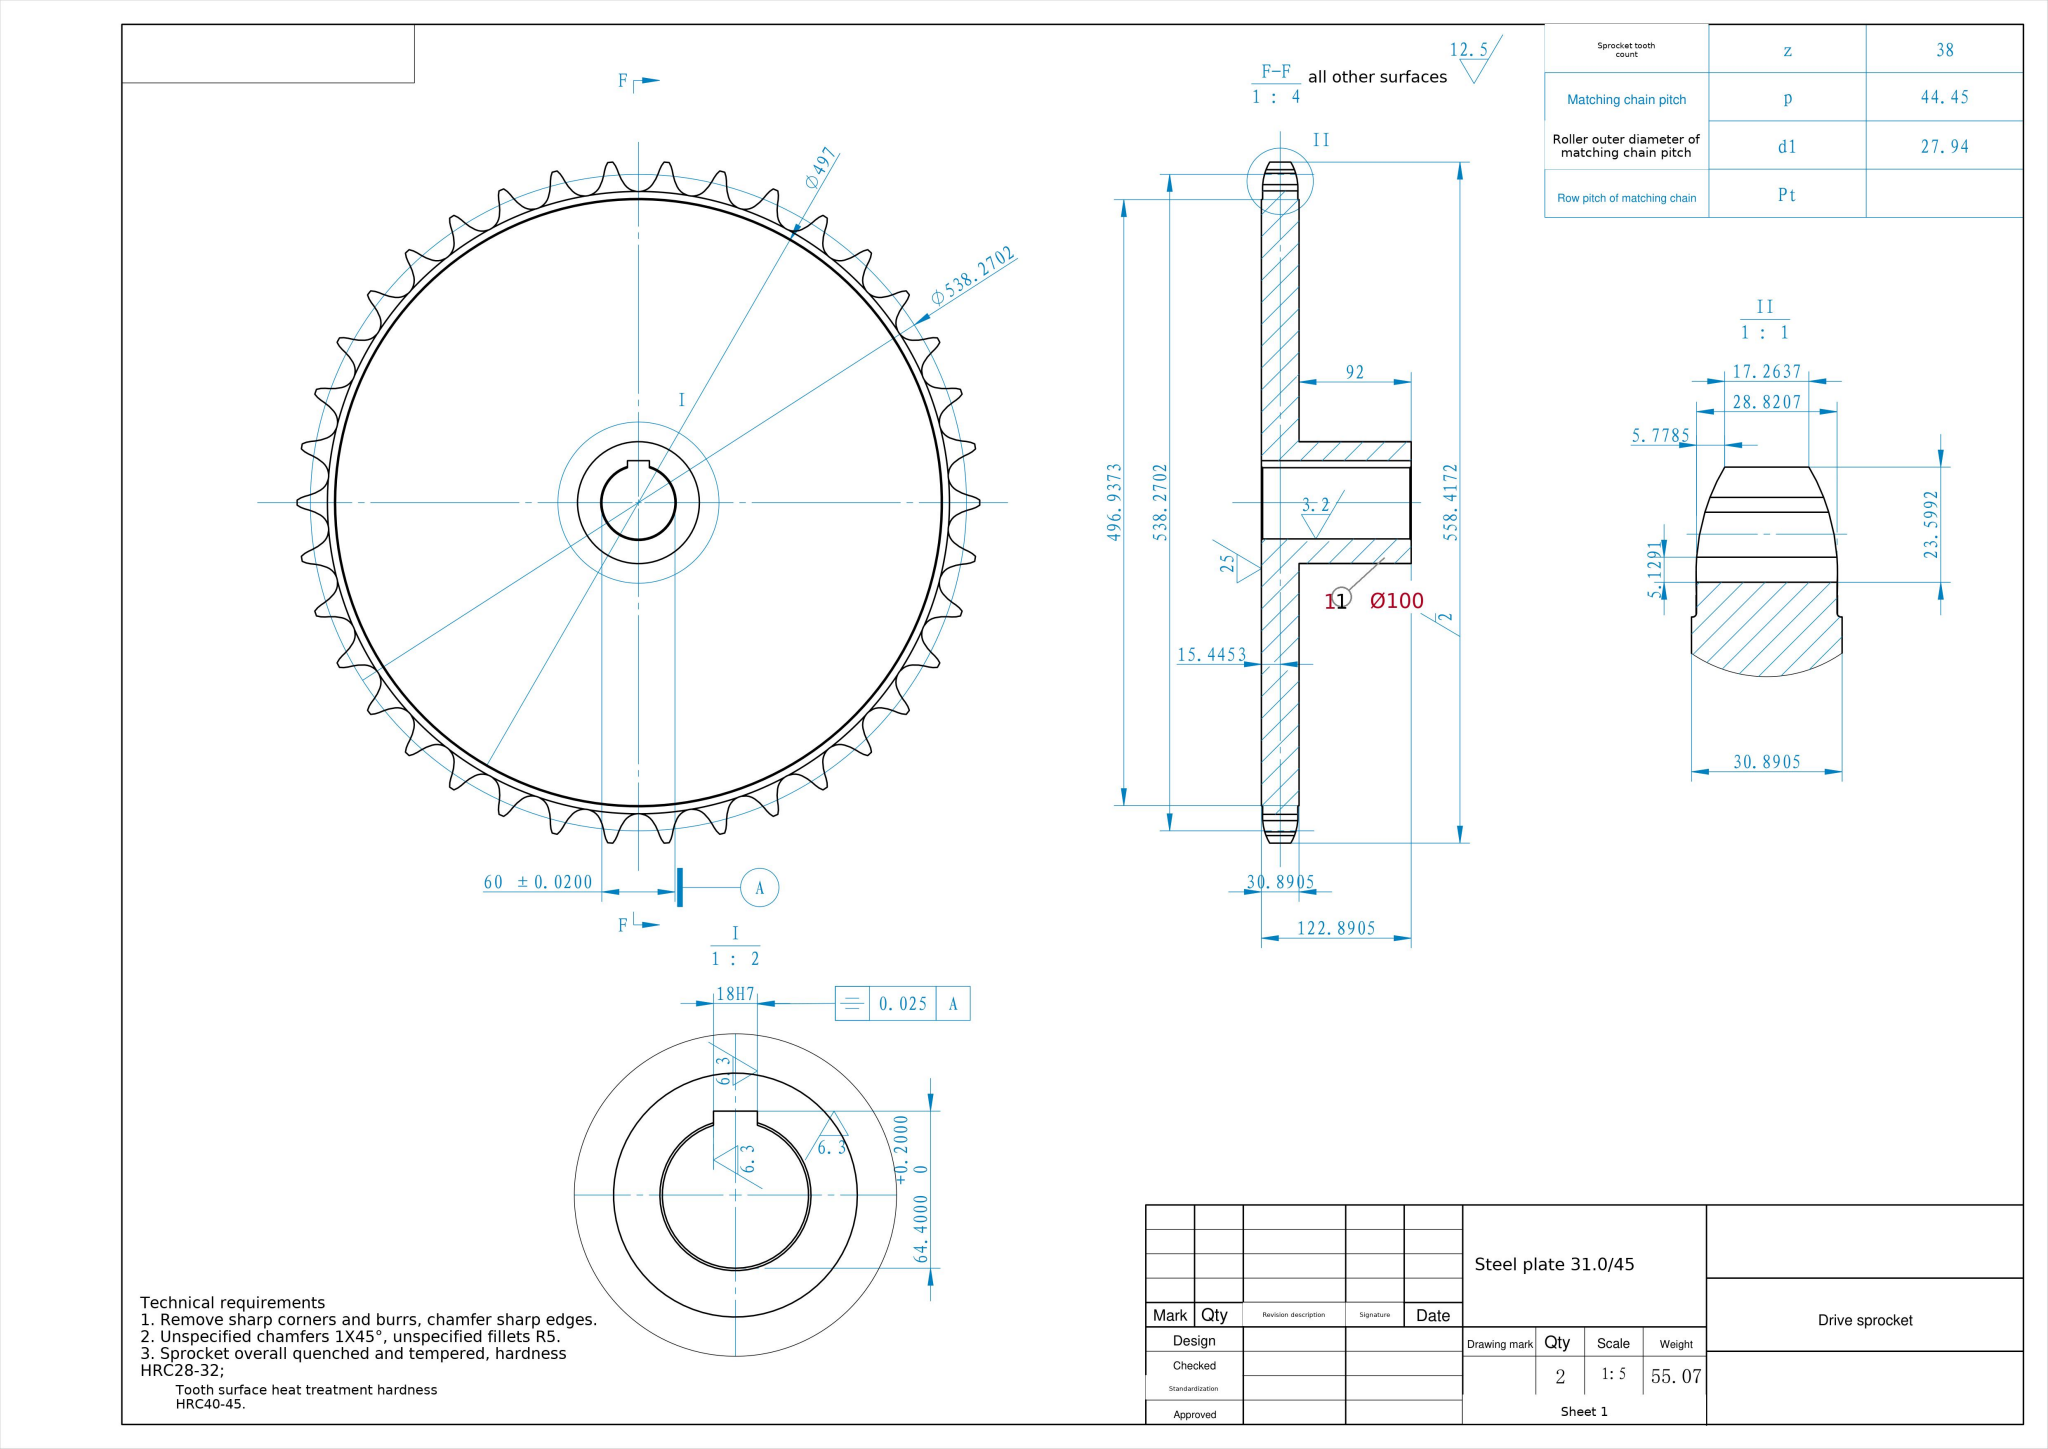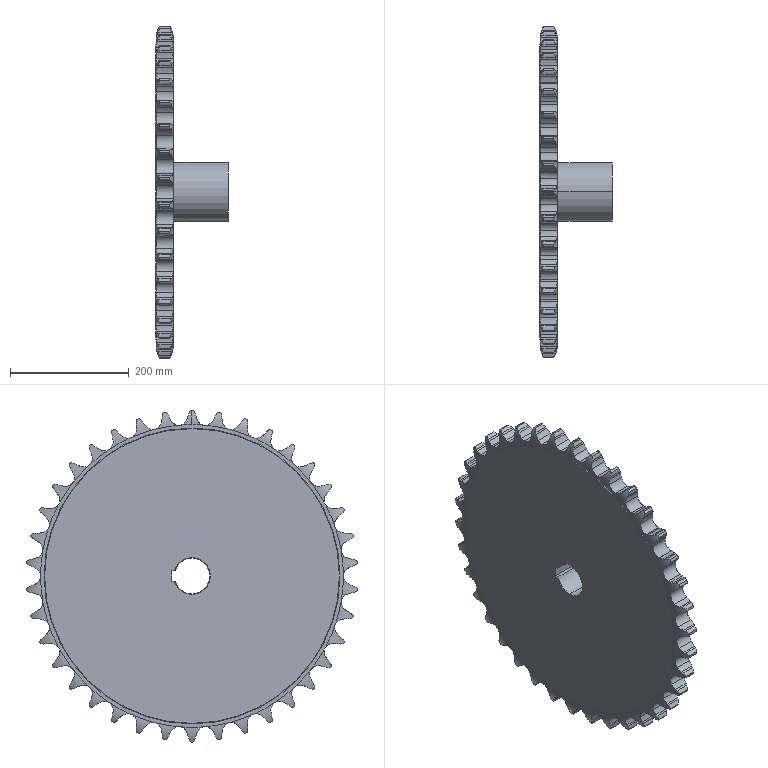Part | SolidWorks | mm | material Steel plate 31.0/45 | 1 solid | 428 faces | box 122.89 x 558.42 x 560 mm | volume 7059989 mm3 | cylinder 256 | plane 84 | torus 82 | cone 6 | commonest cylinder face diameters 40.038 x80 72.884 x78 28.18 x50 560 x39 497 x4 60 x3 100 x2